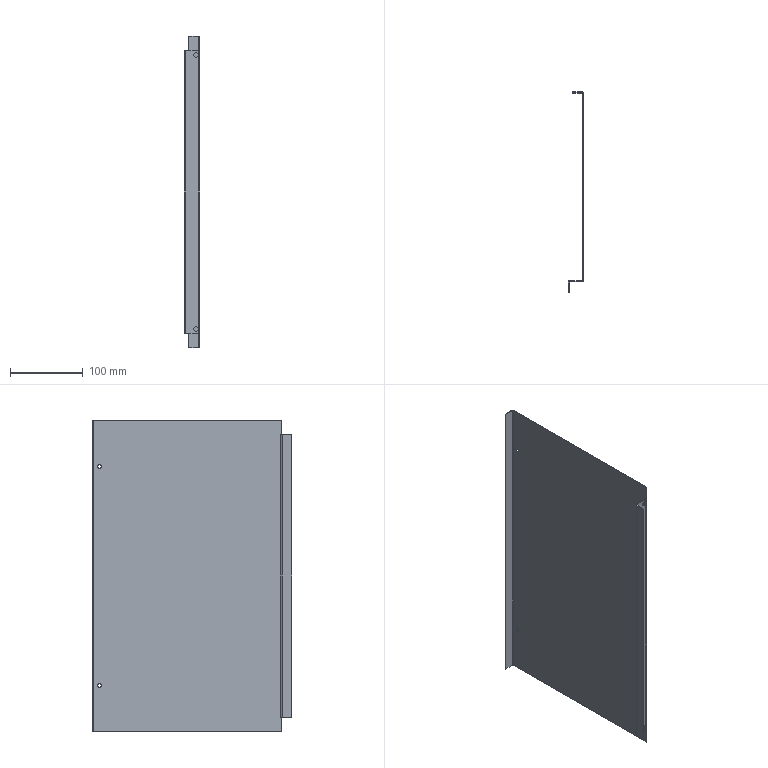Component | SolidWorks | CCQ-1.1-3SideUpperPlate2-2 | 1 solid | 46 faces | volume 129727 mm3 | plane 32 | cylinder 14 | commonest cylinder face diameters 6 x4 5 x4 3.473 x3 1.473 x3 | material 304